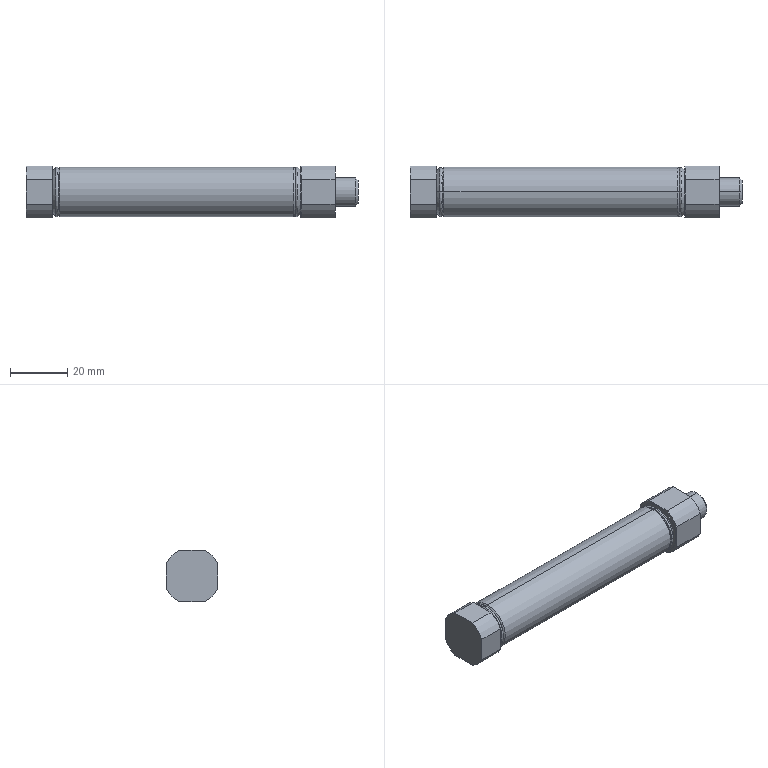Component | SolidWorks | 17268PB16x60SU(58)+(CS1-M-2)-1_1726816PB60UBody-1 | 1 solid | 64 faces | box 116 x 18 x 18 mm | volume 11862 mm3 | cylinder 24 | plane 18 | cone 14 | torus 8 | commonest cylinder face diameters 20 x8 4.134 x4 17.8 x4 16 x2 5 x2 17.4 x2 10 x2
build123d program:
from build123d import *

# Parameters (mm, degrees)
BOSS_EXTRUDE1_DEPTH = 11.8
BOSS_EXTRUDE2_DEPTH = 9.2
HOLE1_D             = 4.134
HOLE1_DEPTH         = 8.1
HOLE1_CSINK_D       = 5
HOLE1_CSINK_ANGLE   = 90
HOLE2_D             = 4.134
HOLE2_DEPTH         = 8.1
HOLE2_CSINK_D       = 5
HOLE2_CSINK_ANGLE   = 90


with BuildPart() as part:
    # Sketch1 → Revolve1 (revolve)
    with BuildSketch(Plane.XY, mode=Mode.PRIVATE) as revolve1_sk:
        Polygon((0, 0), (0, 4.08), (0.92, 5), (8, 5), (8, 0), align=None)
    revolve(revolve1_sk.sketch.rotate(Axis((8, 0, 0), (-1, 0, 0)), 270), axis=Axis((8, 0, 0), (-1, 0, 0)))

    # Sketch2 → Boss-Extrude1 (add)
    with BuildSketch(Plane(origin=(8, 0, 0), x_dir=(0, 0, -1), z_dir=(1, 0, 0))):
        with BuildLine():
            Line((-4.359, -9), (4.359, -9))
            ThreePointArc((4.359, -9), (7.071, -7.071), (9, -4.359))
            Line((9, -4.359), (9, 4.359))
            ThreePointArc((9, 4.359), (7.071, 7.071), (4.359, 9))
            Line((4.359, 9), (-4.359, 9))
            ThreePointArc((-4.359, 9), (-7.071, 7.071), (-9, 4.359))
            Line((-9, 4.359), (-9, -4.359))
            ThreePointArc((-9, -4.359), (-7.071, -7.071), (-4.359, -9))
        make_face()
    extrude(amount=BOSS_EXTRUDE1_DEPTH)

    # Sketch3 → Revolve2 (revolve)
    with BuildSketch(Plane.XY, mode=Mode.PRIVATE) as revolve2_sk:
        with BuildLine():
            Line((19.8, 0), (19.8, 8.9))
            Line((19.8, 8.9), (19.95, 8.9))
            Line((19.95, 8.9), (19.95, 7.62))
            Line((19.95, 7.62), (21.038, 8.533))
            ThreePointArc((21.038, 8.533), (21.403, 8.648), (21.742, 8.471))
            Line((21.742, 8.471), (21.97, 8.2))
            ThreePointArc((21.97, 8.2), (22.157, 8.506), (22.46, 8.7))
            Line((22.46, 8.7), (104.14, 8.7))
            ThreePointArc((104.14, 8.7), (104.443, 8.506), (104.63, 8.2))
            Line((104.63, 8.2), (104.858, 8.471))
            ThreePointArc((104.858, 8.471), (105.197, 8.648), (105.562, 8.533))
            Line((105.562, 8.533), (106.65, 7.62))
            Line((106.65, 7.62), (106.65, 8.9))
            Line((106.65, 8.9), (106.8, 8.9))
            Line((106.8, 8.9), (106.8, 0))
            Line((106.8, 0), (19.8, 0))
        make_face()
    revolve(revolve2_sk.sketch.rotate(Axis((106.8, 0, 0), (-1, 0, 0)), 270), axis=Axis((106.8, 0, 0), (-1, 0, 0)))

    # Sketch4 → Boss-Extrude2 (add)
    with BuildSketch(Plane(origin=(106.8, 0, 0), x_dir=(0, 0, -1), z_dir=(1, 0, 0))):
        with BuildLine():
            Line((-4.359, -9), (4.359, -9))
            ThreePointArc((4.359, -9), (7.071, -7.071), (9, -4.359))
            Line((9, -4.359), (9, 4.359))
            ThreePointArc((9, 4.359), (7.071, 7.071), (4.359, 9))
            Line((4.359, 9), (-4.359, 9))
            ThreePointArc((-4.359, 9), (-7.071, 7.071), (-9, 4.359))
            Line((-9, 4.359), (-9, -4.359))
            ThreePointArc((-9, -4.359), (-7.071, -7.071), (-4.359, -9))
        make_face()
    extrude(amount=BOSS_EXTRUDE2_DEPTH)

    # Hole1
    with Locations(Plane(origin=(0, 9, 0), x_dir=(1, 0, 0), z_dir=(0, 1, 0))):
        with Locations((15.5, 0)):
            CounterSinkHole(HOLE1_D / 2, HOLE1_CSINK_D / 2, depth=HOLE1_DEPTH, counter_sink_angle=HOLE1_CSINK_ANGLE)

    # Hole2
    with Locations(Plane(origin=(0, 9, 0), x_dir=(1, 0, 0), z_dir=(0, 1, 0))):
        with Locations((111.2, 0)):
            CounterSinkHole(HOLE2_D / 2, HOLE2_CSINK_D / 2, depth=HOLE2_DEPTH, counter_sink_angle=HOLE2_CSINK_ANGLE)

    # Sketch9 → Cut-Revolve1 (revolve, cut)
    with BuildSketch(Plane.XY, mode=Mode.PRIVATE) as cut_revolve1_sk:
        Polygon((0, 0), (0, 2.5), (27.16, 2.5), (27.16, 8), (100.36, 8), (100.36, 0), align=None)
    revolve(cut_revolve1_sk.sketch.rotate(Axis((100.36, 0, 0), (-1, 0, 0)), 270), axis=Axis((100.36, 0, 0), (-1, 0, 0)), mode=Mode.SUBTRACT)


solid = part.part

# Placed as in the assembly
solid = solid.moved(Location((-71, -27.579, 21.5), (-180, 0, 180)))